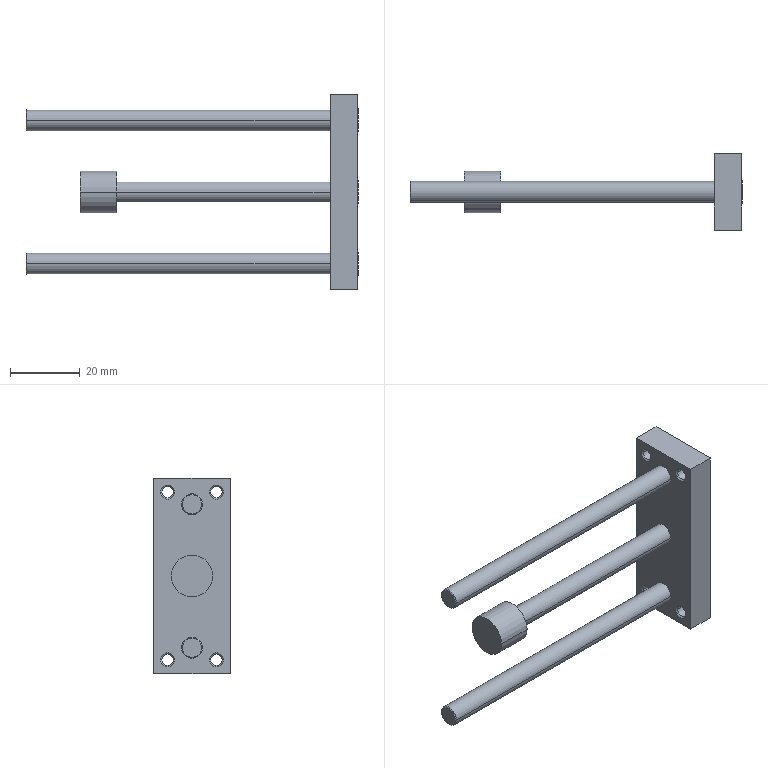Component | SolidWorks | Inline-H010-TCL12x40S_0_+_CS1-G-1-3_Inline-H010-TCL12x40SSteelBallGuide-1 | 1 solid | 89 faces | volume 17222 mm3 | cylinder 34 | cone 34 | plane 21 | commonest cylinder face diameters 6 x12 3.242 x8 3 x6 5.5 x6 11.9 x2